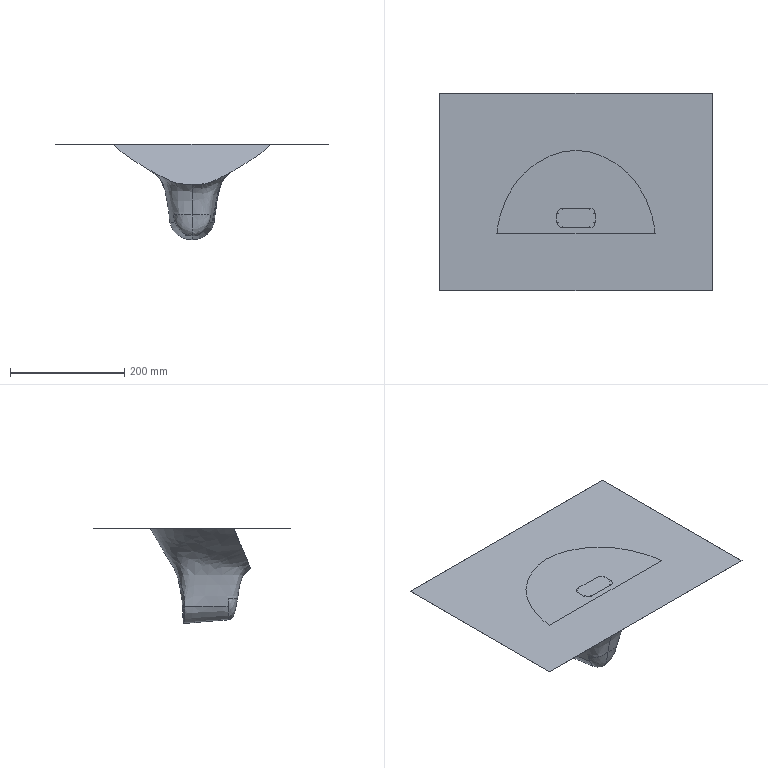CAM job | NX | mm | 3-axis | 1 set-up | 3 operations | part box 477.29 x 346.09 x 167.19
set-up 1
1. Cavity Milling | Mill Mill5 D30R0 | CAVITY_MILL_COPY_COPY_1_COPY_1_COPY | path 236903.22 mm | 46.403 min
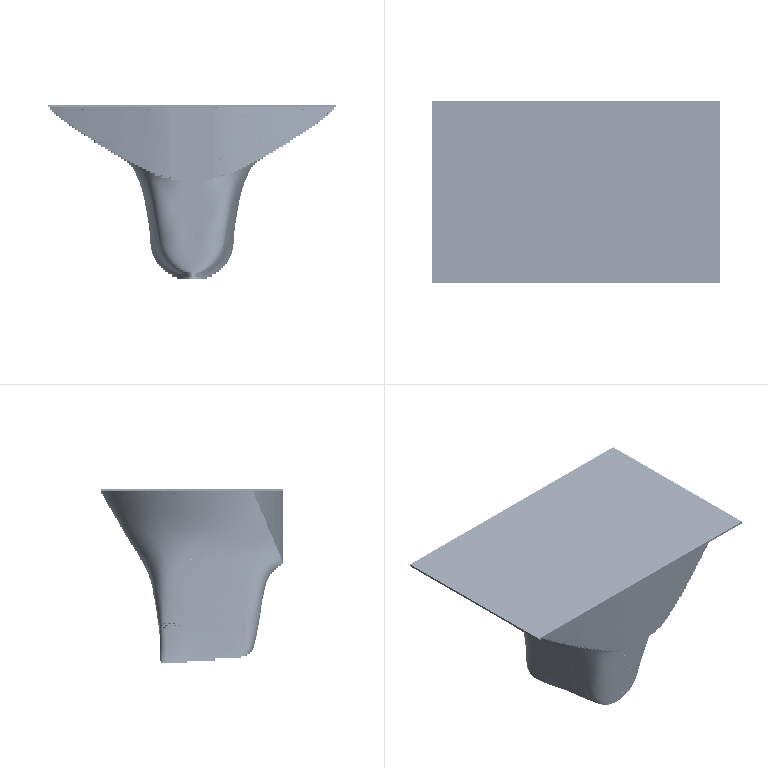2. Z-Level Milling | Mill Mill5 D20R2 | ZLEVEL_PROFILE_COPY_COPY_1 | path 134886.033 mm | 26.747 min
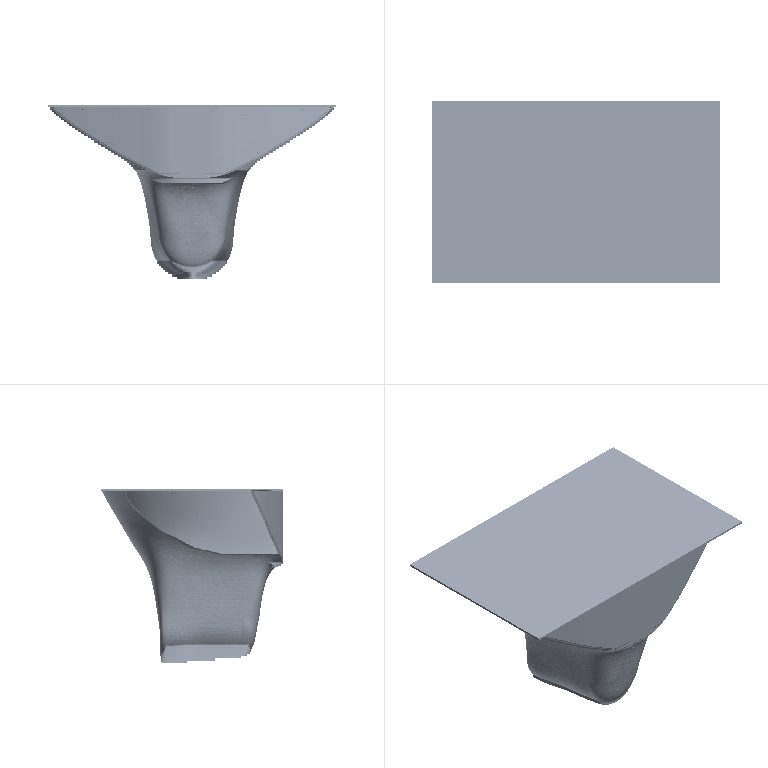3. Fixed-axis Surface Contouring | Mill Mill5 D20R2 | CONTOUR_AREA_COPY_1 | path 114183.973 mm | 22.703 min